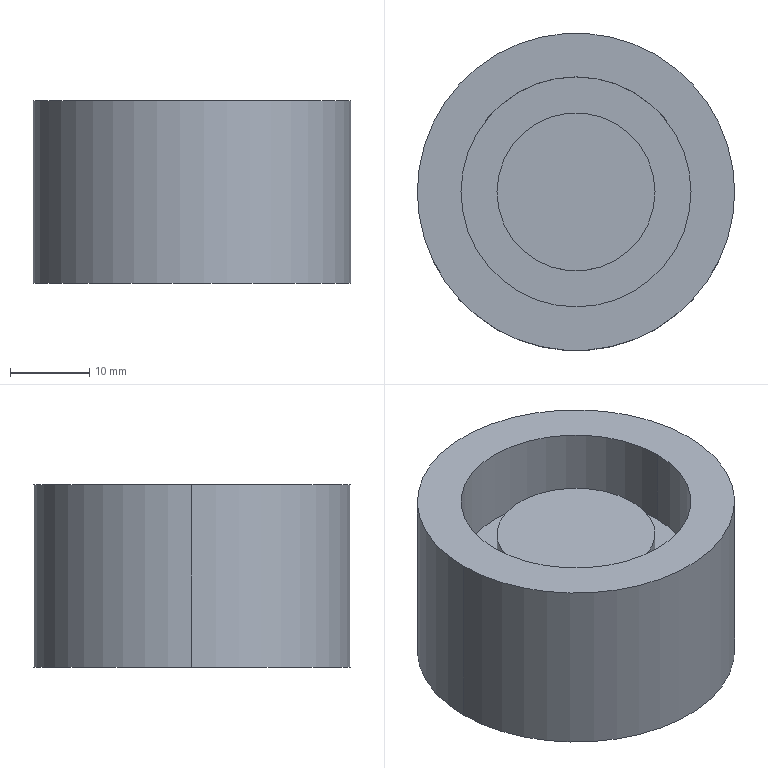CAM job | Mastercam | mm | 7 operations | part box 40 x 40 x 23
1. Pocket (Standard) | 3 - 8 C 平底刀
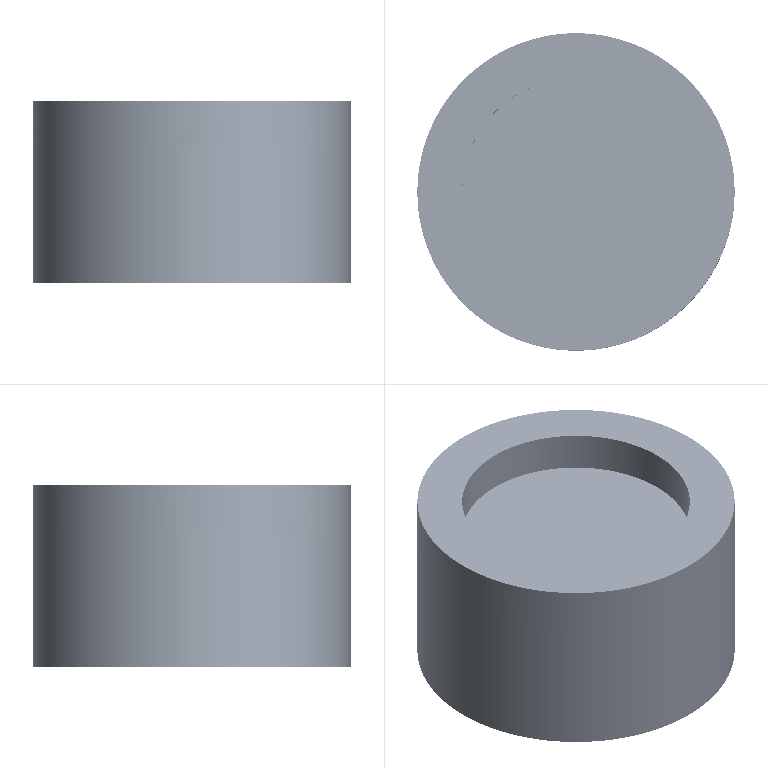2. Circle Mill | 4 - 8 J平底刀
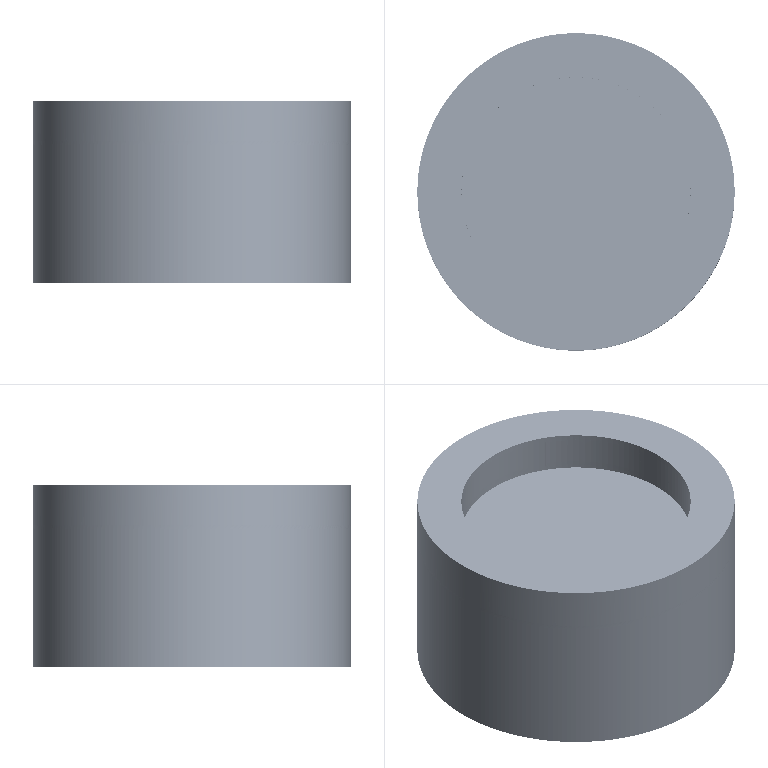3. Contour (Ramp) | 7 - 4 C平底刀
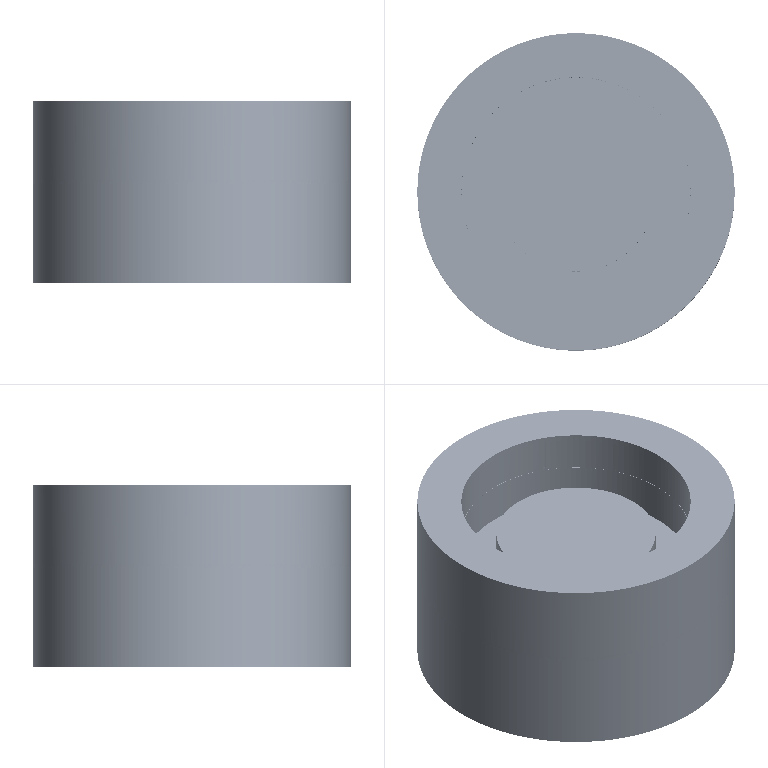4. Circle Mill | 4 - 8 J平底刀
5. Contour (2D) | 8 - 4 J平底刀
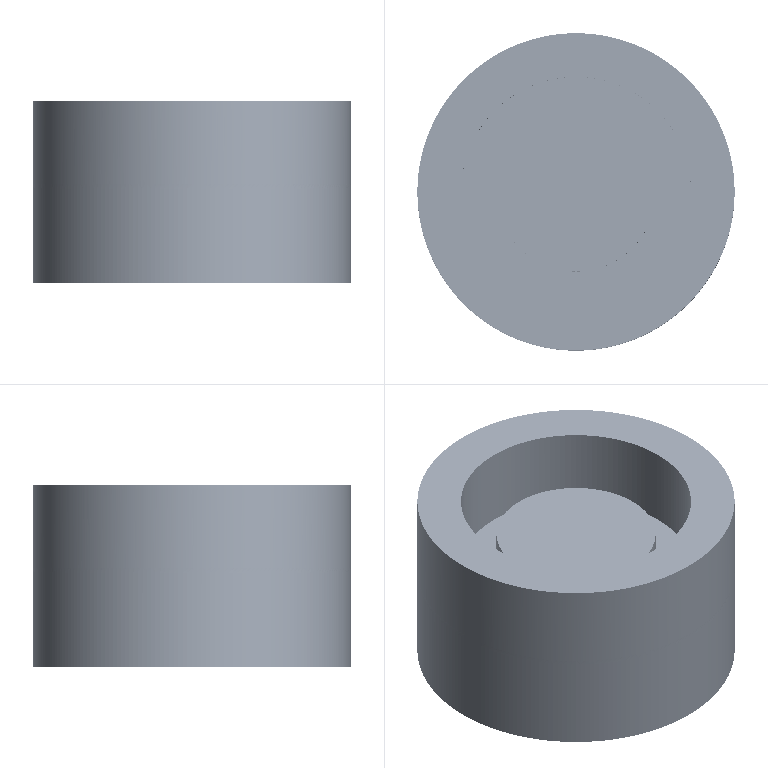6. Contour (2D) | 8 - 4 J平底刀
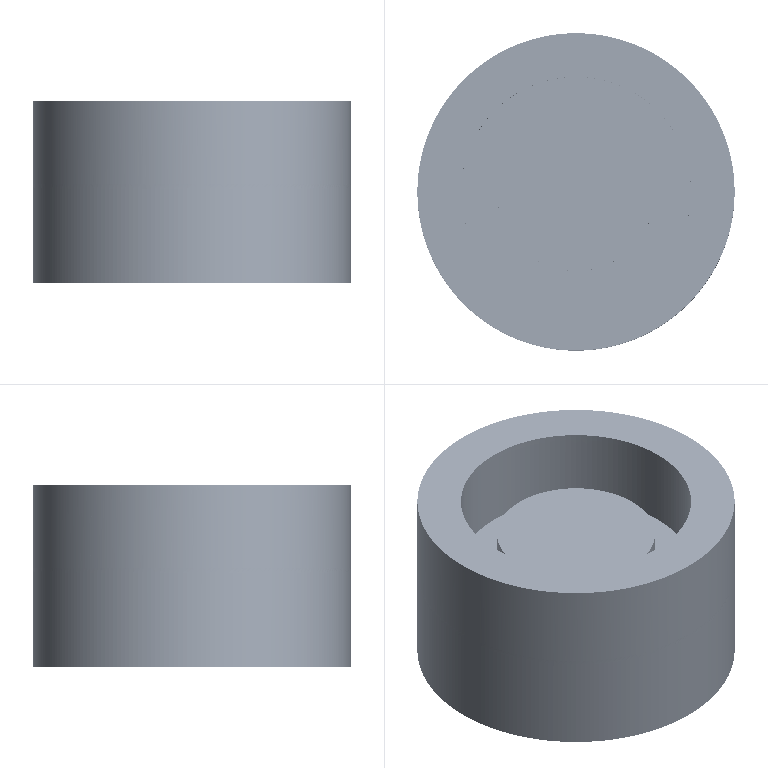7. Model Chamfer | 2 - 6 倒角刀